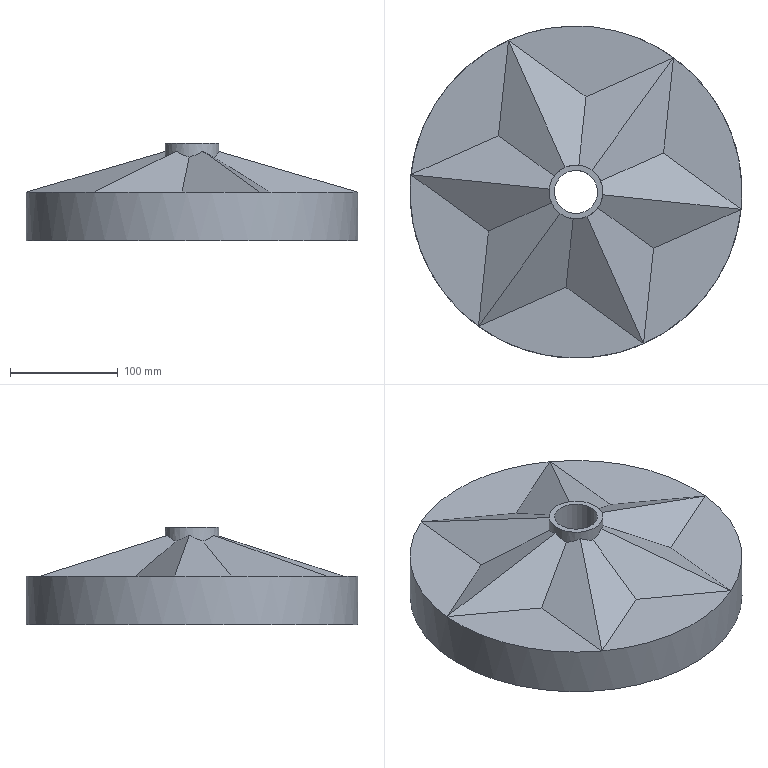Component | NX | ROLLER | 1 solid | 42 faces | volume 3343375 mm3 | plane 35 | cylinder 6 | cone 1 | commonest cylinder face diameters 50 x2 308 x1 40 x1 120 x1 82 x1